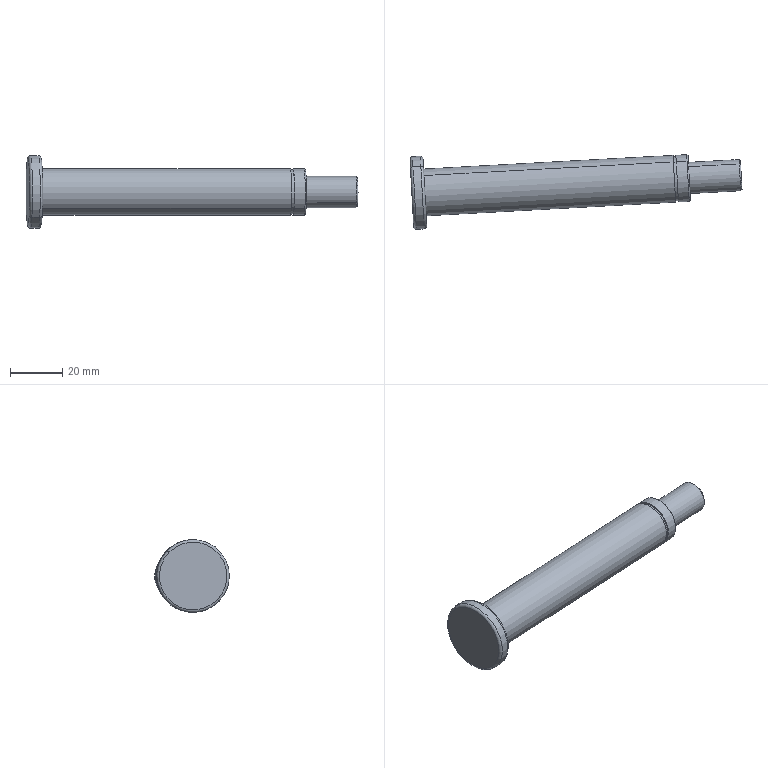Component | SolidWorks | T160418-M01U03-P09-1 | 1 solid | 40 faces | box 127.57 x 28.73 x 28 mm | volume 30365 mm3 | cylinder 18 | plane 12 | cone 6 | torus 4 | commonest cylinder face diameters 4 x6 18 x4 28 x2 17 x2 4.2 x2 12 x2 | material SCr440
build123d program:
from build123d import *

# Parameters (mm, degrees)
SKETCH1_R             = 9
BOSS_EXTRUDE1_DEPTH   = 50.875
SKETCH2_R             = 14
BOSS_EXTRUDE2_DEPTH   = 5
SKETCH5_R             = 6
BOSS_EXTRUDE5_DEPTH   = 20
CUT_EXTRUDE1_START    = 5.5
CUT_EXTRUDE1_DEPTH    = 69.088
M5_TAPPED_HOLE1_D     = 4.2
M5_TAPPED_HOLE1_DEPTH = 14
M5_TAPPED_HOLE1_TIP   = 1.262
CUT_EXTRUDE2_START    = 3.5
CUT_EXTRUDE2_DEPTH    = 71.088
CUT_EXTRUDE3_START    = 96
SKETCH11_OUTSIDE_W    = 56.558
SKETCH11_OUTSIDE_H    = 56.558
SKETCH11_OUTSIDE_R    = 8.5
CUT_EXTRUDE3_DEPTH    = 1.1
FILLET1_R             = 1
CHAMFER1_SIZE         = 0.5


with BuildPart() as part:
    # Sketch1 → Boss-Extrude1 (new, symmetric)
    with BuildSketch(Plane.XY):
        Circle(SKETCH1_R)
    extrude(amount=BOSS_EXTRUDE1_DEPTH, both=True)

    # Sketch2 → Boss-Extrude2 (add)
    with BuildSketch(Plane(origin=(0, 0, -50.875), x_dir=(-1, 0, 0), z_dir=(0, 0, -1))):
        Circle(SKETCH2_R)
    extrude(amount=BOSS_EXTRUDE2_DEPTH)

    # Sketch5 → Boss-Extrude5 (add)
    with BuildSketch(Plane.XY.offset(50.875)):
        Circle(SKETCH5_R)
    extrude(amount=BOSS_EXTRUDE5_DEPTH)

    # Sketch6 → Cut-Extrude1 (cut, through all)
    with BuildSketch(Plane(origin=(0, 0, 0), x_dir=(1, 0, 0), z_dir=(0, 1, 0)).offset(CUT_EXTRUDE1_START)):
        with BuildLine():
            Line((2, 10.875), (2, -19.125))
            ThreePointArc((2, -19.125), (0, -21.125), (-2, -19.125))
            Line((-2, -19.125), (-2, 10.875))
            ThreePointArc((-2, 10.875), (0, 12.875), (2, 10.875))
        make_face()
    extrude(amount=CUT_EXTRUDE1_DEPTH, mode=Mode.SUBTRACT)

    # M5 Tapped Hole1
    with Locations(Plane.XY.offset(70.875)):
        with Locations((0, 0)):
            Hole(M5_TAPPED_HOLE1_D / 2, depth=M5_TAPPED_HOLE1_DEPTH)
            with Locations((0, 0, -(M5_TAPPED_HOLE1_DEPTH + M5_TAPPED_HOLE1_TIP / 2))):  # 118° drill point
                Cone(0, M5_TAPPED_HOLE1_D / 2, M5_TAPPED_HOLE1_TIP, mode=Mode.SUBTRACT)

    # Sketch9 → Cut-Extrude2 (cut, through all)
    with BuildSketch(Plane(origin=(0, 0, 0), x_dir=(1, 0, 0), z_dir=(0, 1, 0)).offset(CUT_EXTRUDE2_START)):
        with BuildLine():
            Line((2, -54.875), (2, -65.875))
            ThreePointArc((2, -65.875), (0, -67.875), (-2, -65.875))
            Line((-2, -65.875), (-2, -54.875))
            ThreePointArc((-2, -54.875), (0, -52.875), (2, -54.875))
        make_face()
    extrude(amount=CUT_EXTRUDE2_DEPTH, mode=Mode.SUBTRACT)

    # Sketch11 outside → Cut-Extrude3 (cut)
    with BuildSketch(Plane.XY.offset(-50.875).offset(CUT_EXTRUDE3_START)):
        Rectangle(SKETCH11_OUTSIDE_W, SKETCH11_OUTSIDE_H)
        Circle(SKETCH11_OUTSIDE_R, mode=Mode.SUBTRACT)
    extrude(amount=CUT_EXTRUDE3_DEPTH, mode=Mode.SUBTRACT)

    # Fillet1
    fillet1_edges = [part.edges().sort_by_distance(p)[0] for p in [
        (14, 0, -50.875),
        (14, 0, -55.875),
    ]]
    fillet(fillet1_edges, radius=FILLET1_R)

    # Chamfer1
    chamfer1_edges = [part.edges().sort_by_distance(p)[0] for p in [
        (-6, 0, 70.875),
        (-9, 0, 50.875),
    ]]
    chamfer(chamfer1_edges, length=CHAMFER1_SIZE)


solid = part.part

# Placed as in the assembly
solid = solid.moved(Location((452.55, 106.198, -217.818), (-90, 86.863, 44.172)))